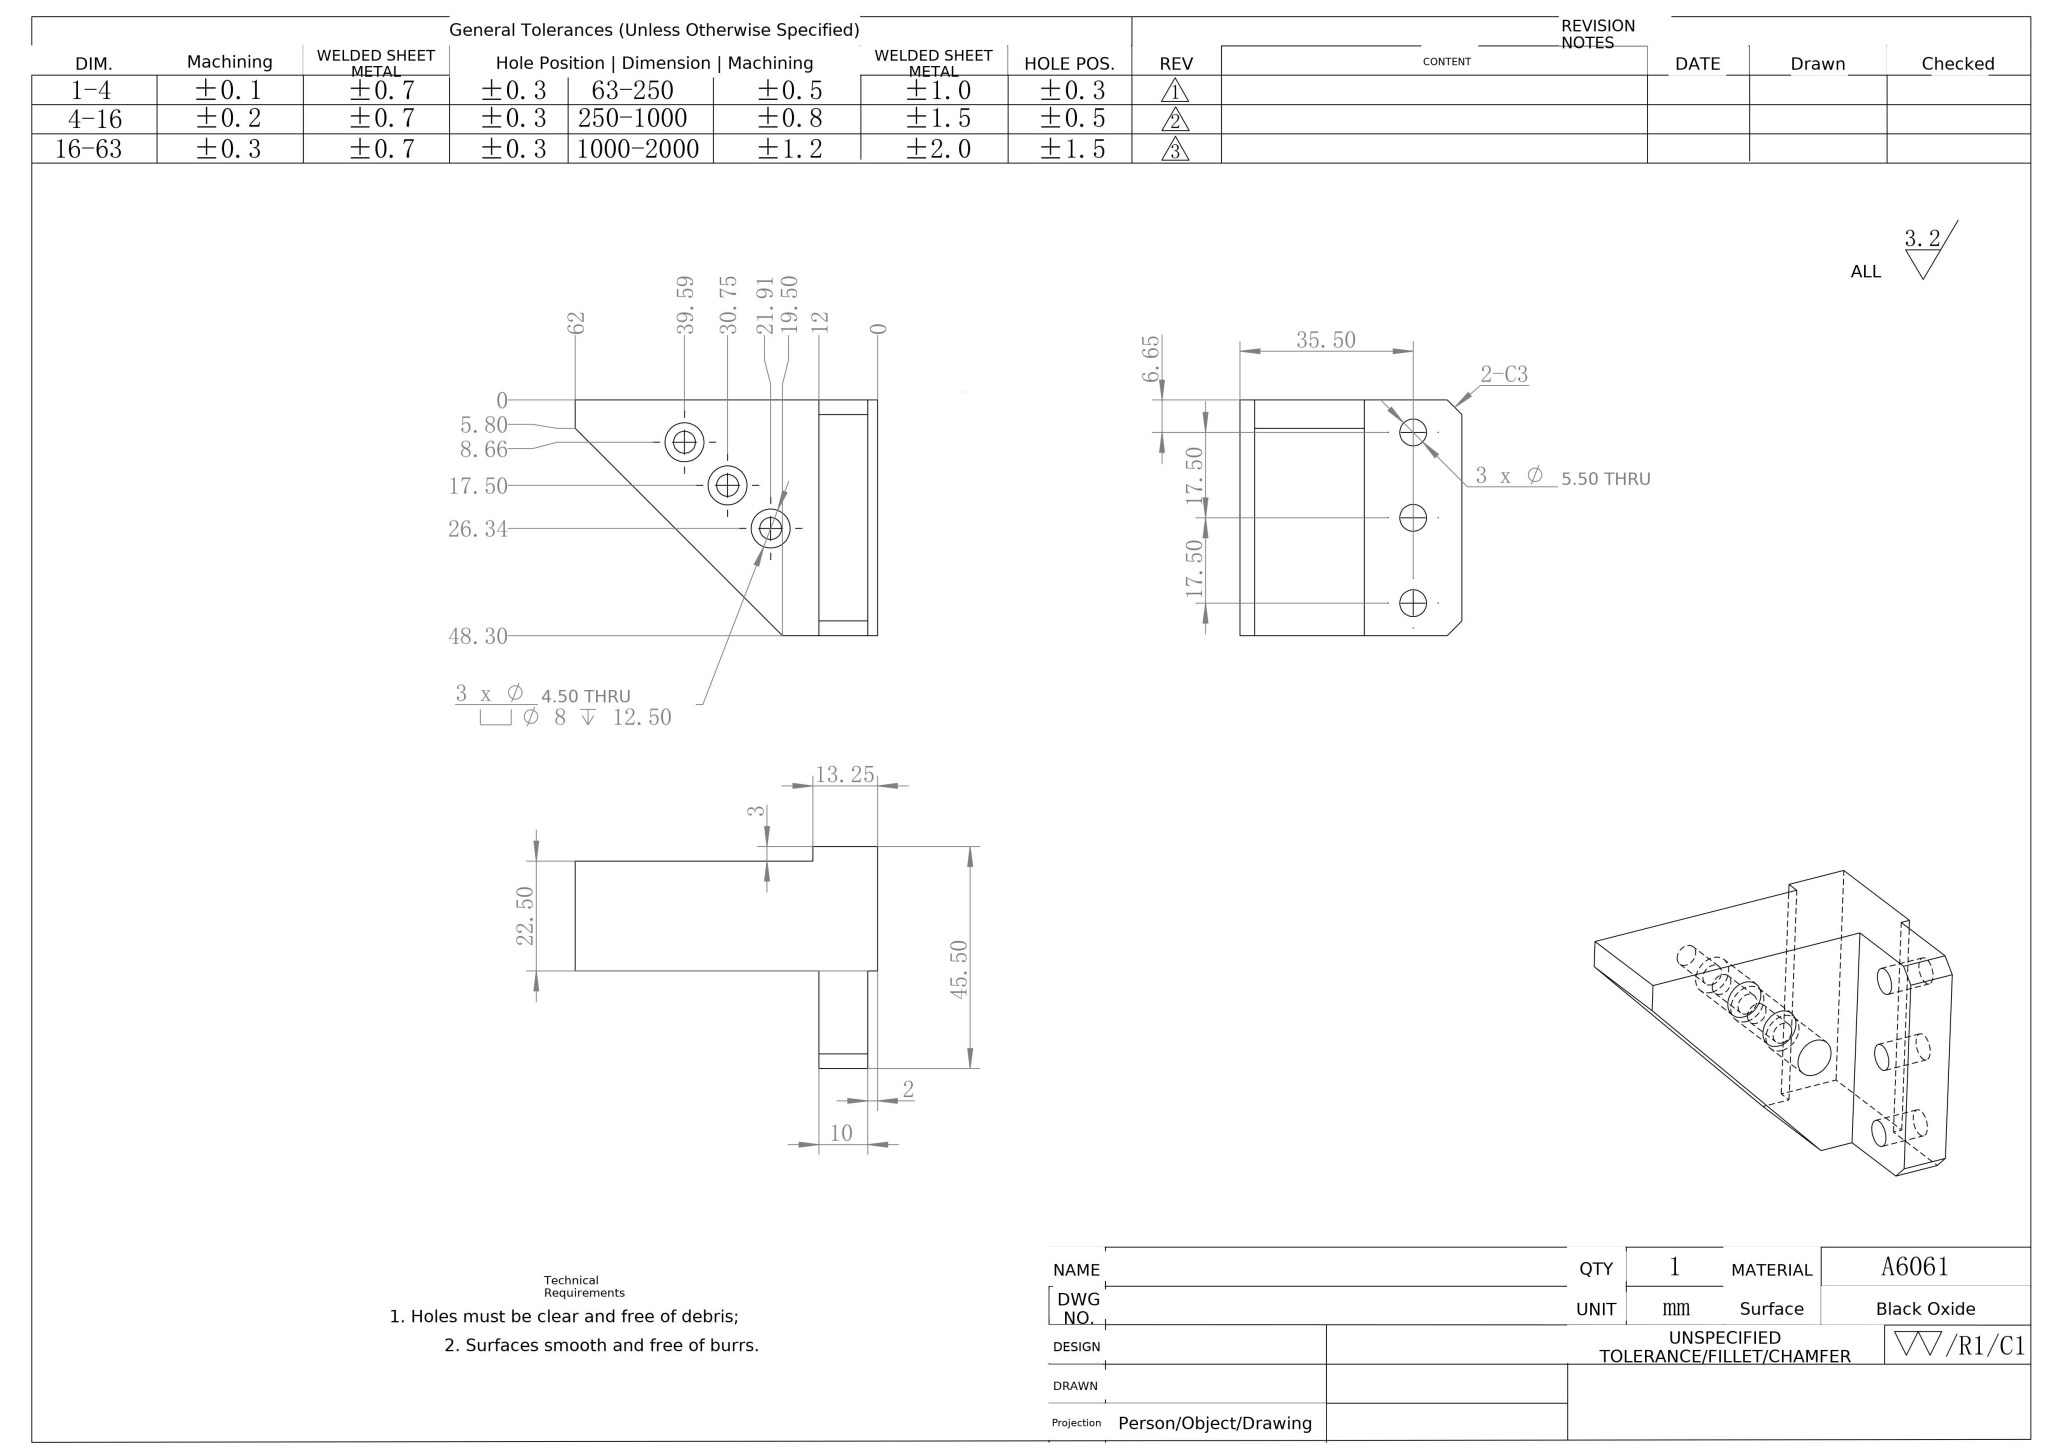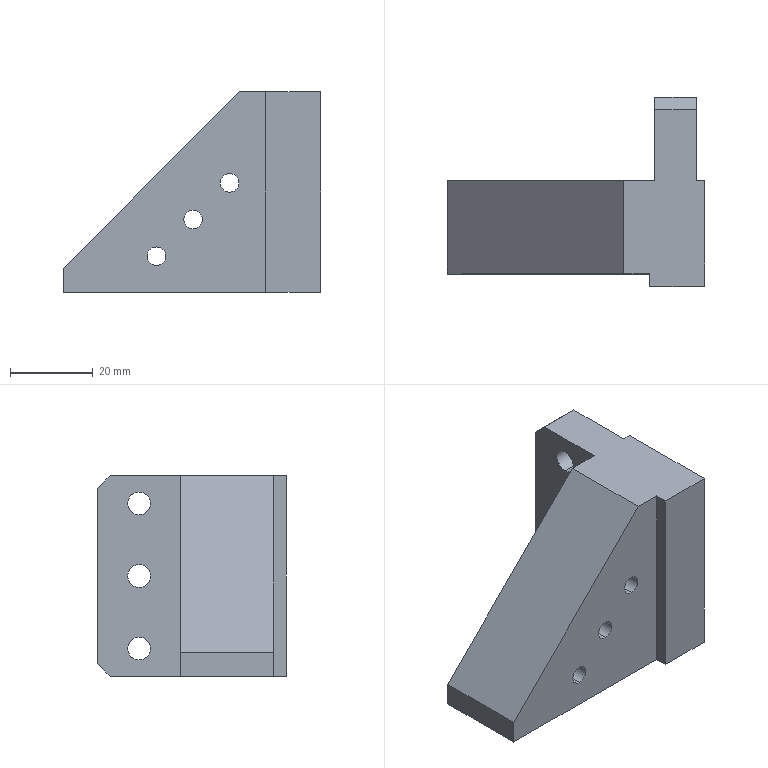Part | NX | mm | Triangular Multi-Bore Corner Bracket | 1 solid | 36 faces | box 62 x 45.5 x 48.3 mm | volume 55473 mm3 | cylinder 18 | plane 18 | commonest cylinder face diameters 5.5 x6 8 x6 4.5 x6